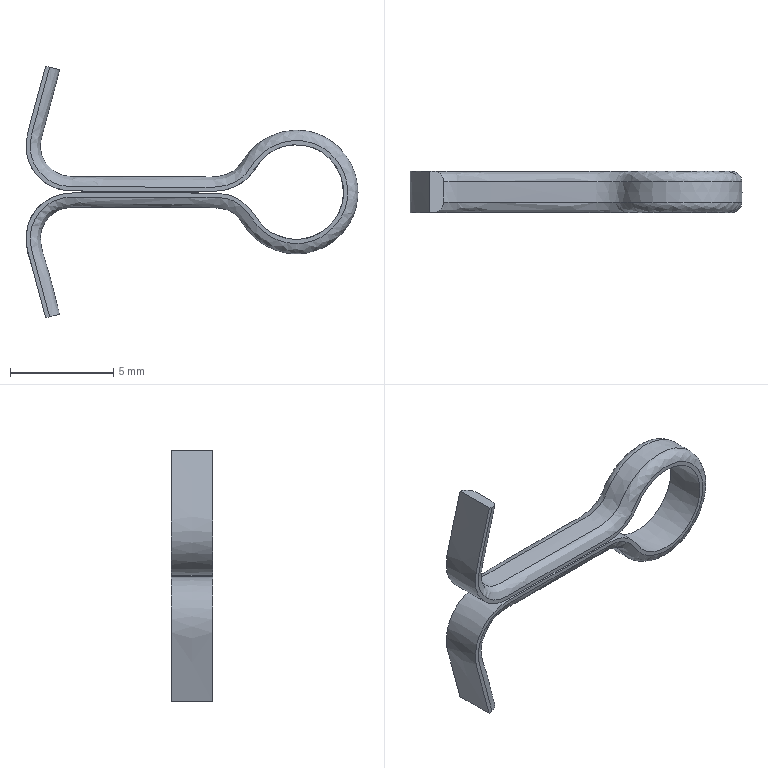Component | NX | QIA | 1 solid | 8 faces | volume 58 mm3 | plane 4 | spline 4